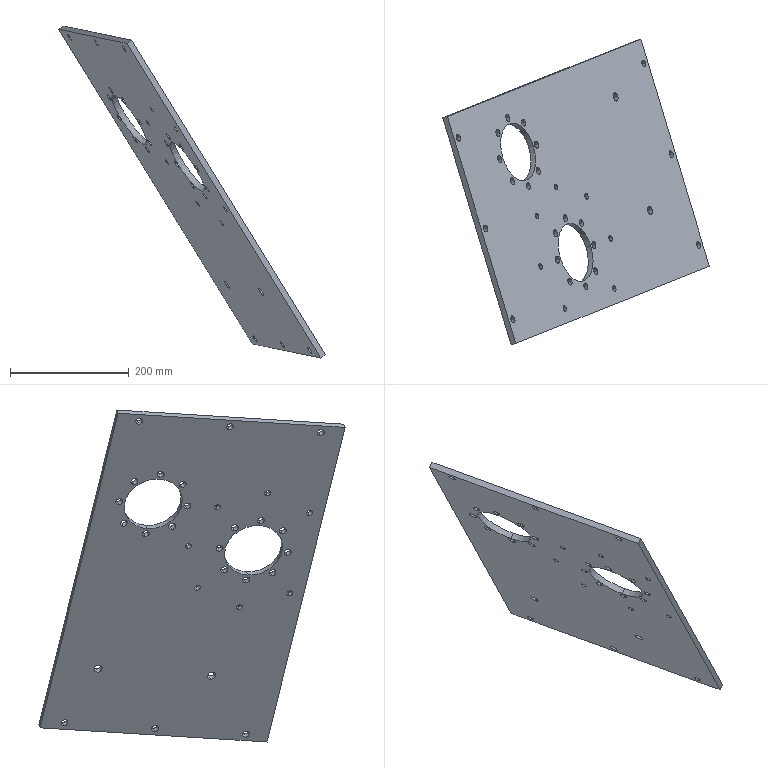Component | SolidWorks | VerticalPlate-2 | 1 solid | 72 faces | box 449.35 x 515.72 x 559.38 mm | volume 2353462 mm3 | cylinder 66 | plane 6 | commonest cylinder face diameters 12 x44 10 x14 14 x4 100 x4
build123d program:
from build123d import *

# Parameters (mm, degrees)
SKETCH1_W          = 760
SKETCH1_H          = 400
EXTRUDE1_DEPTH     = 10
SKETCH2_R          = 50
CUT_EXTRUDE1_DEPTH = 10
SKETCH3_W          = 124
SKETCH3_H          = 400
CUT_EXTRUDE2_DEPTH = 10
SKETCH5_R          = 7
CUT_EXTRUDE3_DEPTH = 10
SKETCH6_R          = 6
CUT_EXTRUDE4_DEPTH = 10
LPATTERN1_COUNT    = 3
LPATTERN1_PITCH    = 160
SKETCH7_R          = 6
CUT_EXTRUDE5_DEPTH = 20
SKETCH8_R          = 5
CUT_EXTRUDE6_DEPTH = 20
CIRPATTERN1_COUNT  = 8
CIRPATTERN2_COUNT  = 8
SKETCH9_R          = 6
CUT_EXTRUDE7_DEPTH = 20
CIRPATTERN3_COUNT  = 8


with BuildPart() as part:
    # Sketch1 → Extrude1 (new body)
    with BuildSketch(Plane.XY):
        with Locations((380, 200)):
            Rectangle(SKETCH1_W, SKETCH1_H)
    extrude(amount=EXTRUDE1_DEPTH)

    # Sketch2 → Cut-Extrude1 (cut)
    with BuildSketch(Plane.XY.offset(10)):
        with Locations((460, 300)):
            Circle(SKETCH2_R)
        with Locations((380, 105.835)):
            Circle(SKETCH2_R)
    extrude(amount=-CUT_EXTRUDE1_DEPTH, mode=Mode.SUBTRACT)

    # Sketch3 → Cut-Extrude2 (cut)
    with BuildSketch(Plane(origin=(0, 0, 0), x_dir=(-1, 0, 0), z_dir=(0, 0, -1))):
        with Locations((-698, 200)):
            Rectangle(SKETCH3_W, SKETCH3_H)
    extrude(amount=-CUT_EXTRUDE2_DEPTH, mode=Mode.SUBTRACT)

    # Sketch5 → Cut-Extrude3 (cut)
    with BuildSketch(Plane.XY.offset(10)):
        with Locations((125, 125)):
            Circle(SKETCH5_R)
        with Locations((125, 325)):
            Circle(SKETCH5_R)
    extrude(amount=-CUT_EXTRUDE3_DEPTH, mode=Mode.SUBTRACT)

    # Sketch6 → Cut-Extrude4 (cut)
    with BuildSketch(Plane(origin=(0, 0, 0), x_dir=(-1, 0, 0), z_dir=(0, 0, -1))):
        with Locations((-623, 360)):
            Circle(SKETCH6_R)
        with Locations(Location((-13, 360, 0), (0, 0, 180))):
            Circle(SKETCH6_R)
    cut_extrude4 = extrude(amount=-CUT_EXTRUDE4_DEPTH, mode=Mode.SUBTRACT)

    # LPattern1: Cut-Extrude4 ×3
    with Locations(*[(0, -i * LPATTERN1_PITCH, 0) for i in range(1, LPATTERN1_COUNT)]):
        add(cut_extrude4, mode=Mode.SUBTRACT)

    # Sketch7 → Cut-Extrude5 (cut)
    with BuildSketch(Plane(origin=(0, 0, 0), x_dir=(-1, 0, 0), z_dir=(0, 0, -1))):
        with Locations((-422.426, 63.409)):
            Circle(SKETCH7_R)
    cut_extrude5 = extrude(amount=-CUT_EXTRUDE5_DEPTH, mode=Mode.SUBTRACT)

    # Sketch8 → Cut-Extrude6 (cut)
    with BuildSketch(Plane(origin=(0, 0, 0), x_dir=(-1, 0, 0), z_dir=(0, 0, -1))):
        with Locations((-461.317, 24.518)):
            Circle(SKETCH8_R)
    cut_extrude6 = extrude(amount=-CUT_EXTRUDE6_DEPTH, mode=Mode.SUBTRACT)

    # CirPattern1: Cut-Extrude5 ×8 about axis
    cirpattern1_axis = Axis((380, 105.835, 0), (0, 0, 1))
    for i in range(1, CIRPATTERN1_COUNT):
        add(cut_extrude5.rotate(cirpattern1_axis, i * 360 / CIRPATTERN1_COUNT), mode=Mode.SUBTRACT)

    # CirPattern2: Cut-Extrude6 ×8 about axis, 1 skipped
    cirpattern2_axis = Axis((380, 105.835, 0), (0, 0, 1))
    add([cut_extrude6.rotate(cirpattern2_axis, i * 360 / CIRPATTERN2_COUNT) for i in range(1, CIRPATTERN2_COUNT) if i not in (7,)], mode=Mode.SUBTRACT)

    # Sketch9 → Cut-Extrude7 (cut)
    with BuildSketch(Plane.XY.offset(10)):
        with Locations((502.426, 342.426)):
            Circle(SKETCH9_R)
    cut_extrude7 = extrude(amount=-CUT_EXTRUDE7_DEPTH, mode=Mode.SUBTRACT)

    # CirPattern3: Cut-Extrude7 ×8 about axis
    cirpattern3_axis = Axis((460, 300, 0), (0, 0, 1))
    for i in range(1, CIRPATTERN3_COUNT):
        add(cut_extrude7.rotate(cirpattern3_axis, i * 360 / CIRPATTERN3_COUNT), mode=Mode.SUBTRACT)


solid = part.part

# Placed as in the assembly
solid = solid.moved(Location((543.724, -191.575, -321.588), (159.138, -53.982, 150.678)))